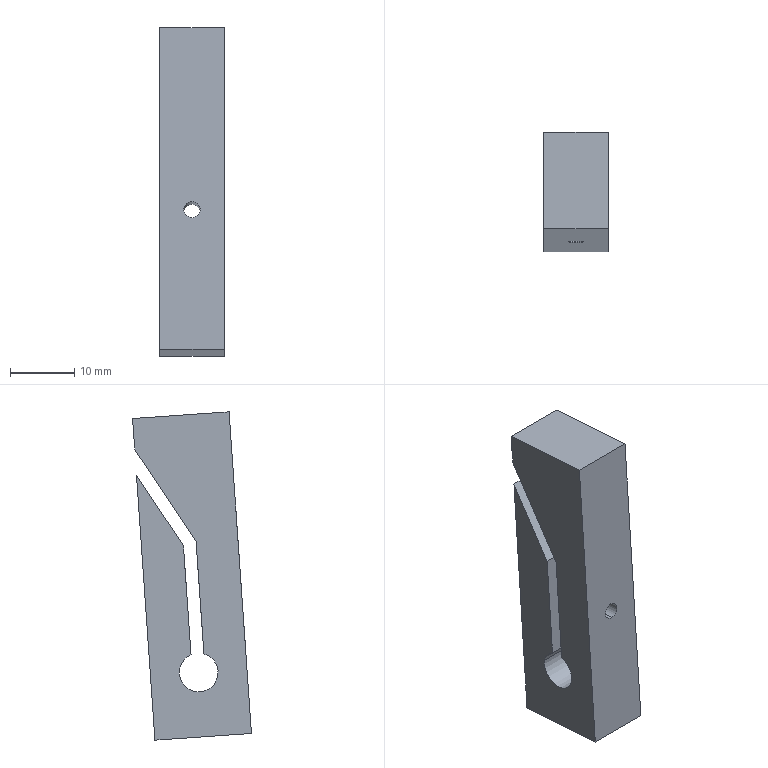Component | SolidWorks | Counterweight-1 | 1 solid | 23 faces | box 10 x 18.44 x 50.92 mm | volume 6250 mm3 | plane 13 | cylinder 8 | cone 2 | commonest cylinder face diameters 4 x3 6 x3 2.5 x2
build123d program:
from build123d import *

# Parameters (mm, degrees)
SKETCH2_R                    = 3
BOSS_EXTRUDE1_DEPTH          = 10
CUT_EXTRUDE_THIN1_DEPTH      = 48.843
CUT_EXTRUDE_THIN1_DEPTH_BACK = 10
CUT_EXTRUDE1_DEPTH           = 8
M3_TAPPED_HOLE1_D            = 2.5
M3_TAPPED_HOLE1_CSINK_D      = 3.05
M3_TAPPED_HOLE1_CSINK_ANGLE  = 90


with BuildPart() as part:
    # Sketch2 → Boss-Extrude1 (new body)
    with BuildSketch(Plane.XY):
        Polygon((1.842, 36.796), (-9.381, -11.928), (-23.998, -8.561), (-12.775, 40.163), align=None)
        with Locations((-14.445, -0.5)):
            Circle(SKETCH2_R, mode=Mode.SUBTRACT)
    extrude(amount=-BOSS_EXTRUDE1_DEPTH)

    # Sketch3 → Cut-Extrude-Thin1 (cut, two sides: drawn at the far end of the back side and taken through both)
    with BuildSketch(Plane.XY.offset(-CUT_EXTRUDE_THIN1_DEPTH_BACK)):
        Polygon((-13.47, -0.7245), (-9.04, 18.508), (2.431, 31.023), (0.9571, 32.375), (-10.871, 19.471), (-15.419, -0.2755), align=None)
    extrude(amount=CUT_EXTRUDE_THIN1_DEPTH + CUT_EXTRUDE_THIN1_DEPTH_BACK, mode=Mode.SUBTRACT)

    # Sketch4 → Cut-Extrude1 (cut)
    with BuildSketch(Plane(origin=(-6.299, 1.451, 0), x_dir=(0, 0, -1), z_dir=(0.9745, -0.2245, 0))):
        with BuildLine():
            Line((7, 12.007), (7, 4.007))
            ThreePointArc((7, 4.007), (5, 2.007), (3, 4.007))
            Line((3, 4.007), (3, 12.007))
            ThreePointArc((3, 12.007), (5, 14.007), (7, 12.007))
        make_face()
    extrude(amount=-CUT_EXTRUDE1_DEPTH, mode=Mode.SUBTRACT)

    # M3 Tapped Hole1 (through all)
    with Locations(Plane(origin=(-14.582, 3.359, 0), x_dir=(0, 0, -1), z_dir=(0.9745, -0.2245, 0))):
        with Locations((5, 8.007)):
            CounterSinkHole(M3_TAPPED_HOLE1_D / 2, M3_TAPPED_HOLE1_CSINK_D / 2, counter_sink_angle=M3_TAPPED_HOLE1_CSINK_ANGLE)


solid = part.part

# Placed as in the assembly
solid = solid.moved(Location((-513.446, 26.616, 404.902), (98.98, 90, 0)))
STEP:
#1=COLOUR_RGB('',0.7922,0.8196,0.9333);
#2=FILL_AREA_STYLE_COLOUR('',#1);
#3=FILL_AREA_STYLE('',(#2));
#4=SURFACE_STYLE_FILL_AREA(#3);
#5=SURFACE_SIDE_STYLE('',(#4));
#6=SURFACE_STYLE_USAGE(.BOTH.,#5);
#7=PRESENTATION_STYLE_ASSIGNMENT((#6));
#8=CARTESIAN_POINT('',(-20.411,0.4679,16.248));
#9=VERTEX_POINT('',#8);
#10=CARTESIAN_POINT('',(-20.411,0.4747,16.346));
#11=VERTEX_POINT('',#10);
#12=CARTESIAN_POINT('',(-20.411,0.4713,16.297));
#13=DIRECTION('',(-0.,0.9976,-0.0696));
#14=DIRECTION('',(0.,0.0696,0.9976));
#15=AXIS2_PLACEMENT_3D('',#12,#13,#14);
#16=CIRCLE('',#15,0.04921);
#17=EDGE_CURVE('',#9,#11,#16,.T.);
#18=ORIENTED_EDGE('',*,*,#17,.F.);
#19=CARTESIAN_POINT('',(-20.411,0.4779,16.237));
#20=VERTEX_POINT('',#19);
#21=CARTESIAN_POINT('',(-20.411,0.4779,16.237));
#22=DIRECTION('',(-0.,0.6562,-0.7546));
#23=VECTOR('',#22,39.37);
#24=LINE('',#21,#23);
#25=EDGE_CURVE('',#9,#20,#24,.T.);
#26=ORIENTED_EDGE('',*,*,#25,.T.);
#27=CARTESIAN_POINT('',(-20.411,0.4863,16.356));
#28=VERTEX_POINT('',#27);
#29=CARTESIAN_POINT('',(-20.411,0.4821,16.296));
#30=DIRECTION('',(-0.,0.9976,-0.0696));
#31=DIRECTION('',(0.,0.0696,0.9976));
#32=AXIS2_PLACEMENT_3D('',#29,#30,#31);
#33=CIRCLE('',#32,0.06004);
#34=EDGE_CURVE('',#20,#28,#33,.T.);
#35=ORIENTED_EDGE('',*,*,#34,.T.);
#36=CARTESIAN_POINT('',(-20.411,0.4863,16.356));
#37=DIRECTION('',(0.,0.7546,0.6562));
#38=VECTOR('',#37,39.37);
#39=LINE('',#36,#38);
#40=EDGE_CURVE('',#11,#28,#39,.T.);
#41=ORIENTED_EDGE('',*,*,#40,.F.);
#42=EDGE_LOOP('',(#18,#26,#35,#41));
#43=FACE_OUTER_BOUND('',#42,.T.);
#44=CARTESIAN_POINT('',(-20.411,0.4821,16.296));
#45=DIRECTION('',(-0.,0.9976,-0.0696));
#46=DIRECTION('',(0.,0.0696,0.9976));
#47=AXIS2_PLACEMENT_3D('',#44,#45,#46);
#48=CONICAL_SURFACE('',#47,0.06004,0.7854);
#49=ADVANCED_FACE('',(#43),#48,.F.);
#50=CARTESIAN_POINT('',(-20.411,0.2303,16.363));
#51=VERTEX_POINT('',#50);
#52=CARTESIAN_POINT('',(-20.411,0.2234,16.265));
#53=VERTEX_POINT('',#52);
#54=CARTESIAN_POINT('',(-20.411,0.2268,16.314));
#55=DIRECTION('',(0.,-0.9976,0.0696));
#56=DIRECTION('',(0.,-0.0696,-0.9976));
#57=AXIS2_PLACEMENT_3D('',#54,#55,#56);
#58=CIRCLE('',#57,0.04921);
#59=EDGE_CURVE('',#51,#53,#58,.T.);
#60=ORIENTED_EDGE('',*,*,#59,.T.);
#61=CARTESIAN_POINT('',(-20.411,0.4787,16.247));
#62=DIRECTION('',(-0.,0.9976,-0.0696));
#63=VECTOR('',#62,39.37);
#64=LINE('',#61,#63);
#65=EDGE_CURVE('',#53,#9,#64,.T.);
#66=ORIENTED_EDGE('',*,*,#65,.T.);
#67=ORIENTED_EDGE('',*,*,#17,.T.);
#68=CARTESIAN_POINT('',(-20.411,0.4855,16.346));
#69=DIRECTION('',(-0.,0.9976,-0.0696));
#70=VECTOR('',#69,39.37);
#71=LINE('',#68,#70);
#72=EDGE_CURVE('',#51,#11,#71,.T.);
#73=ORIENTED_EDGE('',*,*,#72,.F.);
#74=EDGE_LOOP('',(#60,#66,#67,#73));
#75=FACE_OUTER_BOUND('',#74,.T.);
#76=CARTESIAN_POINT('',(-20.411,0.4821,16.296));
#77=DIRECTION('',(-0.,0.9976,-0.0696));
#78=DIRECTION('',(0.,0.0696,0.9976));
#79=AXIS2_PLACEMENT_3D('',#76,#77,#78);
#80=CYLINDRICAL_SURFACE('',#79,0.04921);
#81=ADVANCED_FACE('',(#75),#80,.F.);
#82=CARTESIAN_POINT('',(-20.333,0.5716,16.448));
#83=VERTEX_POINT('',#82);
#84=CARTESIAN_POINT('',(-20.411,0.5771,16.527));
#85=VERTEX_POINT('',#84);
#86=CARTESIAN_POINT('',(-20.411,0.5716,16.448));
#87=DIRECTION('',(0.,-0.9976,0.0696));
#88=DIRECTION('',(0.,-0.0696,-0.9976));
#89=AXIS2_PLACEMENT_3D('',#86,#87,#88);
#90=CIRCLE('',#89,0.07874);
#91=EDGE_CURVE('',#83,#85,#90,.T.);
#92=ORIENTED_EDGE('',*,*,#91,.T.);
#93=CARTESIAN_POINT('',(-20.411,0.8324,16.509));
#94=VERTEX_POINT('',#93);
#95=CARTESIAN_POINT('',(-20.411,0.5182,16.531));
#96=DIRECTION('',(-0.,0.9976,-0.0696));
#97=VECTOR('',#96,39.37);
#98=LINE('',#95,#97);
#99=EDGE_CURVE('',#85,#94,#98,.T.);
#100=ORIENTED_EDGE('',*,*,#99,.T.);
#101=CARTESIAN_POINT('',(-20.333,0.8269,16.43));
#102=VERTEX_POINT('',#101);
#103=CARTESIAN_POINT('',(-20.411,0.8269,16.43));
#104=DIRECTION('',(-0.,0.9976,-0.0696));
#105=DIRECTION('',(0.,0.0696,0.9976));
#106=AXIS2_PLACEMENT_3D('',#103,#104,#105);
#107=CIRCLE('',#106,0.07874);
#108=EDGE_CURVE('',#94,#102,#107,.T.);
#109=ORIENTED_EDGE('',*,*,#108,.T.);
#110=CARTESIAN_POINT('',(-20.333,0.5127,16.452));
#111=DIRECTION('',(-0.,0.9976,-0.0696));
#112=VECTOR('',#111,39.37);
#113=LINE('',#110,#112);
#114=EDGE_CURVE('',#83,#102,#113,.T.);
#115=ORIENTED_EDGE('',*,*,#114,.F.);
#116=EDGE_LOOP('',(#92,#100,#109,#115));
#117=FACE_OUTER_BOUND('',#116,.T.);
#118=CARTESIAN_POINT('',(-20.411,0.5127,16.452));
#119=DIRECTION('',(-0.,0.9976,-0.0696));
#120=DIRECTION('',(0.,0.0696,0.9976));
#121=AXIS2_PLACEMENT_3D('',#118,#119,#120);
#122=CYLINDRICAL_SURFACE('',#121,0.07874);
#123=ADVANCED_FACE('',(#117),#122,.F.);
#124=CARTESIAN_POINT('',(-20.608,0.3726,15.814));
#125=VERTEX_POINT('',#124);
#126=CARTESIAN_POINT('',(-20.608,0.6059,15.851));
#127=VERTEX_POINT('',#126);
#128=CARTESIAN_POINT('',(-20.608,0.4892,15.833));
#129=DIRECTION('',(1.,-0.,-0.));
#130=DIRECTION('',(0.,0.9877,0.1561));
#131=AXIS2_PLACEMENT_3D('',#128,#129,#130);
#132=CIRCLE('',#131,0.1181);
#133=EDGE_CURVE('',#125,#127,#132,.T.);
#134=ORIENTED_EDGE('',*,*,#133,.F.);
#135=CARTESIAN_POINT('',(-20.214,0.3726,15.814));
#136=VERTEX_POINT('',#135);
#137=CARTESIAN_POINT('',(-20.608,0.3726,15.814));
#138=DIRECTION('',(1.,-0.,-0.));
#139=VECTOR('',#138,39.37);
#140=LINE('',#137,#139);
#141=EDGE_CURVE('',#125,#136,#140,.T.);
#142=ORIENTED_EDGE('',*,*,#141,.T.);
#143=CARTESIAN_POINT('',(-20.214,0.6059,15.851));
#144=VERTEX_POINT('',#143);
#145=CARTESIAN_POINT('',(-20.214,0.4892,15.833));
#146=DIRECTION('',(1.,-0.,-0.));
#147=DIRECTION('',(0.,0.9877,0.1561));
#148=AXIS2_PLACEMENT_3D('',#145,#146,#147);
#149=CIRCLE('',#148,0.1181);
#150=EDGE_CURVE('',#136,#144,#149,.T.);
#151=ORIENTED_EDGE('',*,*,#150,.T.);
#152=CARTESIAN_POINT('',(-20.608,0.6059,15.851));
#153=DIRECTION('',(1.,-0.,-0.));
#154=VECTOR('',#153,39.37);
#155=LINE('',#152,#154);
#156=EDGE_CURVE('',#127,#144,#155,.T.);
#157=ORIENTED_EDGE('',*,*,#156,.F.);
#158=EDGE_LOOP('',(#134,#142,#151,#157));
#159=FACE_OUTER_BOUND('',#158,.T.);
#160=CARTESIAN_POINT('',(-20.608,0.4892,15.833));
#161=DIRECTION('',(1.,-0.,-0.));
#162=DIRECTION('',(0.,0.9877,0.1561));
#163=AXIS2_PLACEMENT_3D('',#160,#161,#162);
#164=CYLINDRICAL_SURFACE('',#163,0.1181);
#165=ADVANCED_FACE('',(#159),#164,.F.);
#166=CARTESIAN_POINT('',(-20.608,0.5363,15.941));
#167=VERTEX_POINT('',#166);
#168=CARTESIAN_POINT('',(-20.608,0.4892,15.833));
#169=DIRECTION('',(1.,-0.,-0.));
#170=DIRECTION('',(0.,0.9877,0.1561));
#171=AXIS2_PLACEMENT_3D('',#168,#169,#170);
#172=CIRCLE('',#171,0.1181);
#173=EDGE_CURVE('',#127,#167,#172,.T.);
#174=ORIENTED_EDGE('',*,*,#173,.F.);
#175=ORIENTED_EDGE('',*,*,#156,.T.);
#176=CARTESIAN_POINT('',(-20.214,0.5363,15.941));
#177=VERTEX_POINT('',#176);
#178=CARTESIAN_POINT('',(-20.214,0.4892,15.833));
#179=DIRECTION('',(1.,-0.,-0.));
#180=DIRECTION('',(0.,0.9877,0.1561));
#181=AXIS2_PLACEMENT_3D('',#178,#179,#180);
#182=CIRCLE('',#181,0.1181);
#183=EDGE_CURVE('',#144,#177,#182,.T.);
#184=ORIENTED_EDGE('',*,*,#183,.T.);
#185=CARTESIAN_POINT('',(-20.608,0.5363,15.941));
#186=DIRECTION('',(1.,-0.,-0.));
#187=VECTOR('',#186,39.37);
#188=LINE('',#185,#187);
#189=EDGE_CURVE('',#167,#177,#188,.T.);
#190=ORIENTED_EDGE('',*,*,#189,.F.);
#191=EDGE_LOOP('',(#174,#175,#184,#190));
#192=FACE_OUTER_BOUND('',#191,.T.);
#193=CARTESIAN_POINT('',(-20.608,0.4892,15.833));
#194=DIRECTION('',(1.,-0.,-0.));
#195=DIRECTION('',(0.,0.9877,0.1561));
#196=AXIS2_PLACEMENT_3D('',#193,#194,#195);
#197=CYLINDRICAL_SURFACE('',#196,0.1181);
#198=ADVANCED_FACE('',(#192),#197,.F.);
#199=CARTESIAN_POINT('',(-20.49,0.8269,16.43));
#200=VERTEX_POINT('',#199);
#201=CARTESIAN_POINT('',(-20.411,0.8269,16.43));
#202=DIRECTION('',(-0.,0.9976,-0.0696));
#203=DIRECTION('',(0.,0.0696,0.9976));
#204=AXIS2_PLACEMENT_3D('',#201,#202,#203);
#205=CIRCLE('',#204,0.07874);
#206=EDGE_CURVE('',#200,#94,#205,.T.);
#207=ORIENTED_EDGE('',*,*,#206,.F.);
#208=CARTESIAN_POINT('',(-20.49,0.805,16.116));
#209=VERTEX_POINT('',#208);
#210=CARTESIAN_POINT('',(-20.49,0.8269,16.43));
#211=DIRECTION('',(0.,0.0696,0.9976));
#212=VECTOR('',#211,39.37);
#213=LINE('',#210,#212);
#214=EDGE_CURVE('',#209,#200,#213,.T.);
#215=ORIENTED_EDGE('',*,*,#214,.F.);
#216=CARTESIAN_POINT('',(-20.333,0.805,16.116));
#217=VERTEX_POINT('',#216);
#218=CARTESIAN_POINT('',(-20.411,0.805,16.116));
#219=DIRECTION('',(-0.,0.9976,-0.0696));
#220=DIRECTION('',(0.,0.0696,0.9976));
#221=AXIS2_PLACEMENT_3D('',#218,#219,#220);
#222=CIRCLE('',#221,0.07874);
#223=EDGE_CURVE('',#217,#209,#222,.T.);
#224=ORIENTED_EDGE('',*,*,#223,.F.);
#225=CARTESIAN_POINT('',(-20.333,0.8269,16.43));
#226=DIRECTION('',(-0.,-0.0696,-0.9976));
#227=VECTOR('',#226,39.37);
#228=LINE('',#225,#227);
#229=EDGE_CURVE('',#102,#217,#228,.T.);
#230=ORIENTED_EDGE('',*,*,#229,.F.);
#231=ORIENTED_EDGE('',*,*,#108,.F.);
#232=EDGE_LOOP('',(#207,#215,#224,#230,#231));
#233=FACE_BOUND('',#232,.T.);
#234=CARTESIAN_POINT('',(-20.608,0.7564,15.42));
#235=VERTEX_POINT('',#234);
#236=CARTESIAN_POINT('',(-20.608,0.8693,17.038));
#237=VERTEX_POINT('',#236);
#238=CARTESIAN_POINT('',(-20.608,0.8934,17.383));
#239=DIRECTION('',(0.,0.0696,0.9976));
#240=VECTOR('',#239,39.37);
#241=LINE('',#238,#240);
#242=EDGE_CURVE('',#235,#237,#241,.T.);
#243=ORIENTED_EDGE('',*,*,#242,.T.);
#244=CARTESIAN_POINT('',(-20.214,0.8693,17.038));
#245=VERTEX_POINT('',#244);
#246=CARTESIAN_POINT('',(-20.608,0.8693,17.038));
#247=DIRECTION('',(1.,-0.,-0.));
#248=VECTOR('',#247,39.37);
#249=LINE('',#246,#248);
#250=EDGE_CURVE('',#237,#245,#249,.T.);
#251=ORIENTED_EDGE('',*,*,#250,.T.);
#252=CARTESIAN_POINT('',(-20.214,0.7564,15.42));
#253=VERTEX_POINT('',#252);
#254=CARTESIAN_POINT('',(-20.214,0.8934,17.383));
#255=DIRECTION('',(0.,0.0696,0.9976));
#256=VECTOR('',#255,39.37);
#257=LINE('',#254,#256);
#258=EDGE_CURVE('',#253,#245,#257,.T.);
#259=ORIENTED_EDGE('',*,*,#258,.F.);
#260=CARTESIAN_POINT('',(-20.608,0.7564,15.42));
#261=DIRECTION('',(1.,-0.,-0.));
#262=VECTOR('',#261,39.37);
#263=LINE('',#260,#262);
#264=EDGE_CURVE('',#235,#253,#263,.T.);
#265=ORIENTED_EDGE('',*,*,#264,.F.);
#266=EDGE_LOOP('',(#243,#251,#259,#265));
#267=FACE_OUTER_BOUND('',#266,.T.);
#268=CARTESIAN_POINT('',(-20.608,0.8934,17.383));
#269=DIRECTION('',(-0.,0.9976,-0.0696));
#270=DIRECTION('',(0.,0.0696,0.9976));
#271=AXIS2_PLACEMENT_3D('',#268,#269,#270);
#272=PLANE('',#271);
#273=ADVANCED_FACE('',(#233,#267),#272,.T.);
#274=CARTESIAN_POINT('',(-20.214,0.8934,17.383));
#275=VERTEX_POINT('',#274);
#276=CARTESIAN_POINT('',(-20.214,0.3043,17.424));
#277=VERTEX_POINT('',#276);
#278=CARTESIAN_POINT('',(-20.214,0.3043,17.424));
#279=DIRECTION('',(0.,-0.9976,0.0696));
#280=VECTOR('',#279,39.37);
#281=LINE('',#278,#280);
#282=EDGE_CURVE('',#275,#277,#281,.T.);
#283=ORIENTED_EDGE('',*,*,#282,.F.);
#284=CARTESIAN_POINT('',(-20.608,0.8934,17.383));
#285=VERTEX_POINT('',#284);
#286=CARTESIAN_POINT('',(-20.608,0.8934,17.383));
#287=DIRECTION('',(1.,-0.,-0.));
#288=VECTOR('',#287,39.37);
#289=LINE('',#286,#288);
#290=EDGE_CURVE('',#285,#275,#289,.T.);
#291=ORIENTED_EDGE('',*,*,#290,.F.);
#292=CARTESIAN_POINT('',(-20.608,0.3043,17.424));
#293=VERTEX_POINT('',#292);
#294=CARTESIAN_POINT('',(-20.608,0.3043,17.424));
#295=DIRECTION('',(0.,-0.9976,0.0696));
#296=VECTOR('',#295,39.37);
#297=LINE('',#294,#296);
#298=EDGE_CURVE('',#285,#293,#297,.T.);
#299=ORIENTED_EDGE('',*,*,#298,.T.);
#300=CARTESIAN_POINT('',(-20.608,0.3043,17.424));
#301=DIRECTION('',(1.,-0.,-0.));
#302=VECTOR('',#301,39.37);
#303=LINE('',#300,#302);
#304=EDGE_CURVE('',#293,#277,#303,.T.);
#305=ORIENTED_EDGE('',*,*,#304,.T.);
#306=EDGE_LOOP('',(#283,#291,#299,#305));
#307=FACE_OUTER_BOUND('',#306,.T.);
#308=CARTESIAN_POINT('',(-20.608,0.3043,17.424));
#309=DIRECTION('',(0.,0.0696,0.9976));
#310=DIRECTION('',(0.,-0.9976,0.0696));
#311=AXIS2_PLACEMENT_3D('',#308,#309,#310);
#312=PLANE('',#311);
#313=ADVANCED_FACE('',(#307),#312,.T.);
#314=CARTESIAN_POINT('',(-20.608,0.8804,17.197));
#315=VERTEX_POINT('',#314);
#316=CARTESIAN_POINT('',(-20.214,0.8804,17.197));
#317=VERTEX_POINT('',#316);
#318=CARTESIAN_POINT('',(-20.608,0.8804,17.197));
#319=DIRECTION('',(1.,-0.,-0.));
#320=VECTOR('',#319,39.37);
#321=LINE('',#318,#320);
#322=EDGE_CURVE('',#315,#317,#321,.T.);
#323=ORIENTED_EDGE('',*,*,#322,.F.);
#324=CARTESIAN_POINT('',(-20.608,0.8934,17.383));
#325=DIRECTION('',(0.,0.0696,0.9976));
#326=VECTOR('',#325,39.37);
#327=LINE('',#324,#326);
#328=EDGE_CURVE('',#315,#285,#327,.T.);
#329=ORIENTED_EDGE('',*,*,#328,.T.);
#330=ORIENTED_EDGE('',*,*,#290,.T.);
#331=CARTESIAN_POINT('',(-20.214,0.8934,17.383));
#332=DIRECTION('',(0.,0.0696,0.9976));
#333=VECTOR('',#332,39.37);
#334=LINE('',#331,#333);
#335=EDGE_CURVE('',#317,#275,#334,.T.);
#336=ORIENTED_EDGE('',*,*,#335,.F.);
#337=EDGE_LOOP('',(#323,#329,#330,#336));
#338=FACE_OUTER_BOUND('',#337,.T.);
#339=CARTESIAN_POINT('',(-20.608,0.8934,17.383));
#340=DIRECTION('',(-0.,0.9976,-0.0696));
#341=DIRECTION('',(0.,0.0696,0.9976));
#342=AXIS2_PLACEMENT_3D('',#339,#340,#341);
#343=PLANE('',#342);
#344=ADVANCED_FACE('',(#338),#343,.T.);
#345=CARTESIAN_POINT('',(-20.214,0.1673,15.461));
#346=VERTEX_POINT('',#345);
#347=CARTESIAN_POINT('',(-20.214,0.7564,15.42));
#348=DIRECTION('',(-0.,0.9976,-0.0696));
#349=VECTOR('',#348,39.37);
#350=LINE('',#347,#349);
#351=EDGE_CURVE('',#346,#253,#350,.T.);
#352=ORIENTED_EDGE('',*,*,#351,.F.);
#353=CARTESIAN_POINT('',(-20.608,0.1673,15.461));
#354=VERTEX_POINT('',#353);
#355=CARTESIAN_POINT('',(-20.608,0.1673,15.461));
#356=DIRECTION('',(1.,-0.,-0.));
#357=VECTOR('',#356,39.37);
#358=LINE('',#355,#357);
#359=EDGE_CURVE('',#354,#346,#358,.T.);
#360=ORIENTED_EDGE('',*,*,#359,.F.);
#361=CARTESIAN_POINT('',(-20.608,0.7564,15.42));
#362=DIRECTION('',(-0.,0.9976,-0.0696));
#363=VECTOR('',#362,39.37);
#364=LINE('',#361,#363);
#365=EDGE_CURVE('',#354,#235,#364,.T.);
#366=ORIENTED_EDGE('',*,*,#365,.T.);
#367=ORIENTED_EDGE('',*,*,#264,.T.);
#368=EDGE_LOOP('',(#352,#360,#366,#367));
#369=FACE_OUTER_BOUND('',#368,.T.);
#370=CARTESIAN_POINT('',(-20.608,0.7564,15.42));
#371=DIRECTION('',(-0.,-0.0696,-0.9976));
#372=DIRECTION('',(-0.,0.9976,-0.0696));
#373=AXIS2_PLACEMENT_3D('',#370,#371,#372);
#374=PLANE('',#373);
#375=ADVANCED_FACE('',(#369),#374,.T.);
#376=ORIENTED_EDGE('',*,*,#59,.F.);
#377=CARTESIAN_POINT('',(-20.411,0.2268,16.314));
#378=DIRECTION('',(0.,-0.9976,0.0696));
#379=DIRECTION('',(0.,-0.0696,-0.9976));
#380=AXIS2_PLACEMENT_3D('',#377,#378,#379);
#381=CIRCLE('',#380,0.04921);
#382=EDGE_CURVE('',#53,#51,#381,.T.);
#383=ORIENTED_EDGE('',*,*,#382,.F.);
#384=EDGE_LOOP('',(#376,#383));
#385=FACE_BOUND('',#384,.T.);
#386=CARTESIAN_POINT('',(-20.214,0.1673,15.461));
#387=DIRECTION('',(-0.,-0.0696,-0.9976));
#388=VECTOR('',#387,39.37);
#389=LINE('',#386,#388);
#390=EDGE_CURVE('',#277,#346,#389,.T.);
#391=ORIENTED_EDGE('',*,*,#390,.F.);
#392=ORIENTED_EDGE('',*,*,#304,.F.);
#393=CARTESIAN_POINT('',(-20.608,0.1673,15.461));
#394=DIRECTION('',(-0.,-0.0696,-0.9976));
#395=VECTOR('',#394,39.37);
#396=LINE('',#393,#395);
#397=EDGE_CURVE('',#293,#354,#396,.T.);
#398=ORIENTED_EDGE('',*,*,#397,.T.);
#399=ORIENTED_EDGE('',*,*,#359,.T.);
#400=EDGE_LOOP('',(#391,#392,#398,#399));
#401=FACE_OUTER_BOUND('',#400,.T.);
#402=CARTESIAN_POINT('',(-20.608,0.1673,15.461));
#403=DIRECTION('',(0.,-0.9976,0.0696));
#404=DIRECTION('',(-0.,-0.0696,-0.9976));
#405=AXIS2_PLACEMENT_3D('',#402,#403,#404);
#406=PLANE('',#405);
#407=ADVANCED_FACE('',(#385,#401),#406,.T.);
#408=CARTESIAN_POINT('',(-20.608,0.5055,16.631));
#409=VERTEX_POINT('',#408);
#410=CARTESIAN_POINT('',(-20.608,0.5112,16.64));
#411=DIRECTION('',(0.,0.5524,0.8336));
#412=VECTOR('',#411,39.37);
#413=LINE('',#410,#412);
#414=EDGE_CURVE('',#409,#315,#413,.T.);
#415=ORIENTED_EDGE('',*,*,#414,.F.);
#416=CARTESIAN_POINT('',(-20.608,0.4577,15.947));
#417=VERTEX_POINT('',#416);
#418=CARTESIAN_POINT('',(-20.608,0.45,15.836));
#419=DIRECTION('',(0.,0.0696,0.9976));
#420=VECTOR('',#419,39.37);
#421=LINE('',#418,#420);
#422=EDGE_CURVE('',#417,#409,#421,.T.);
#423=ORIENTED_EDGE('',*,*,#422,.F.);
#424=CARTESIAN_POINT('',(-20.608,0.4892,15.833));
#425=DIRECTION('',(1.,-0.,-0.));
#426=DIRECTION('',(0.,0.9877,0.1561));
#427=AXIS2_PLACEMENT_3D('',#424,#425,#426);
#428=CIRCLE('',#427,0.1181);
#429=EDGE_CURVE('',#417,#125,#428,.T.);
#430=ORIENTED_EDGE('',*,*,#429,.T.);
#431=ORIENTED_EDGE('',*,*,#133,.T.);
#432=ORIENTED_EDGE('',*,*,#173,.T.);
#433=CARTESIAN_POINT('',(-20.608,0.5826,16.605));
#434=VERTEX_POINT('',#433);
#435=CARTESIAN_POINT('',(-20.608,0.5285,15.83));
#436=DIRECTION('',(0.,0.0696,0.9976));
#437=VECTOR('',#436,39.37);
#438=LINE('',#435,#437);
#439=EDGE_CURVE('',#167,#434,#438,.T.);
#440=ORIENTED_EDGE('',*,*,#439,.T.);
#441=CARTESIAN_POINT('',(-20.608,0.5769,16.597));
#442=DIRECTION('',(0.,0.5524,0.8336));
#443=VECTOR('',#442,39.37);
#444=LINE('',#441,#443);
#445=EDGE_CURVE('',#434,#237,#444,.T.);
#446=ORIENTED_EDGE('',*,*,#445,.T.);
#447=ORIENTED_EDGE('',*,*,#242,.F.);
#448=ORIENTED_EDGE('',*,*,#365,.F.);
#449=ORIENTED_EDGE('',*,*,#397,.F.);
#450=ORIENTED_EDGE('',*,*,#298,.F.);
#451=ORIENTED_EDGE('',*,*,#328,.F.);
#452=EDGE_LOOP('',(#415,#423,#430,#431,#432,#440,#446,#447,#448,#449,#450,#451));
#453=FACE_OUTER_BOUND('',#452,.T.);
#454=CARTESIAN_POINT('',(-20.608,1.048,15.941));
#455=DIRECTION('',(-1.,0.,0.));
#456=DIRECTION('',(-0.,-0.9877,-0.1561));
#457=AXIS2_PLACEMENT_3D('',#454,#455,#456);
#458=PLANE('',#457);
#459=ADVANCED_FACE('',(#453),#458,.T.);
#460=CARTESIAN_POINT('',(-20.214,0.4577,15.947));
#461=VERTEX_POINT('',#460);
#462=CARTESIAN_POINT('',(-20.214,0.5055,16.631));
#463=VERTEX_POINT('',#462);
#464=CARTESIAN_POINT('',(-20.214,0.4602,15.982));
#465=DIRECTION('',(0.,0.0696,0.9976));
#466=VECTOR('',#465,39.37);
#467=LINE('',#464,#466);
#468=EDGE_CURVE('',#461,#463,#467,.T.);
#469=ORIENTED_EDGE('',*,*,#468,.T.);
#470=CARTESIAN_POINT('',(-20.214,0.3531,16.401));
#471=DIRECTION('',(0.,0.5524,0.8336));
#472=VECTOR('',#471,39.37);
#473=LINE('',#470,#472);
#474=EDGE_CURVE('',#463,#317,#473,.T.);
#475=ORIENTED_EDGE('',*,*,#474,.T.);
#476=ORIENTED_EDGE('',*,*,#335,.T.);
#477=ORIENTED_EDGE('',*,*,#282,.T.);
#478=ORIENTED_EDGE('',*,*,#390,.T.);
#479=ORIENTED_EDGE('',*,*,#351,.T.);
#480=ORIENTED_EDGE('',*,*,#258,.T.);
#481=CARTESIAN_POINT('',(-20.214,0.5826,16.605));
#482=VERTEX_POINT('',#481);
#483=CARTESIAN_POINT('',(-20.214,0.4187,16.358));
#484=DIRECTION('',(0.,0.5524,0.8336));
#485=VECTOR('',#484,39.37);
#486=LINE('',#483,#485);
#487=EDGE_CURVE('',#482,#245,#486,.T.);
#488=ORIENTED_EDGE('',*,*,#487,.F.);
#489=CARTESIAN_POINT('',(-20.214,0.5387,15.977));
#490=DIRECTION('',(0.,0.0696,0.9976));
#491=VECTOR('',#490,39.37);
#492=LINE('',#489,#491);
#493=EDGE_CURVE('',#177,#482,#492,.T.);
#494=ORIENTED_EDGE('',*,*,#493,.F.);
#495=ORIENTED_EDGE('',*,*,#183,.F.);
#496=ORIENTED_EDGE('',*,*,#150,.F.);
#497=CARTESIAN_POINT('',(-20.214,0.4892,15.833));
#498=DIRECTION('',(1.,-0.,-0.));
#499=DIRECTION('',(0.,0.9877,0.1561));
#500=AXIS2_PLACEMENT_3D('',#497,#498,#499);
#501=CIRCLE('',#500,0.1181);
#502=EDGE_CURVE('',#461,#136,#501,.T.);
#503=ORIENTED_EDGE('',*,*,#502,.F.);
#504=EDGE_LOOP('',(#469,#475,#476,#477,#478,#479,#480,#488,#494,#495,#496,#503));
#505=FACE_OUTER_BOUND('',#504,.T.);
#506=CARTESIAN_POINT('',(-20.214,1.048,15.941));
#507=DIRECTION('',(-1.,0.,0.));
#508=DIRECTION('',(-0.,-0.9877,-0.1561));
#509=AXIS2_PLACEMENT_3D('',#506,#507,#508);
#510=PLANE('',#509);
#511=ADVANCED_FACE('',(#505),#510,.F.);
#512=ORIENTED_EDGE('',*,*,#141,.F.);
#513=ORIENTED_EDGE('',*,*,#429,.F.);
#514=CARTESIAN_POINT('',(-20.608,0.4577,15.947));
#515=DIRECTION('',(1.,-0.,-0.));
#516=VECTOR('',#515,39.37);
#517=LINE('',#514,#516);
#518=EDGE_CURVE('',#417,#461,#517,.T.);
#519=ORIENTED_EDGE('',*,*,#518,.T.);
#520=ORIENTED_EDGE('',*,*,#502,.T.);
#521=EDGE_LOOP('',(#512,#513,#519,#520));
#522=FACE_OUTER_BOUND('',#521,.T.);
#523=CARTESIAN_POINT('',(-20.608,0.4892,15.833));
#524=DIRECTION('',(1.,-0.,-0.));
#525=DIRECTION('',(0.,0.9877,0.1561));
#526=AXIS2_PLACEMENT_3D('',#523,#524,#525);
#527=CYLINDRICAL_SURFACE('',#526,0.1181);
#528=ADVANCED_FACE('',(#522),#527,.F.);
#529=ORIENTED_EDGE('',*,*,#91,.F.);
#530=CARTESIAN_POINT('',(-20.333,0.5497,16.134));
#531=VERTEX_POINT('',#530);
#532=CARTESIAN_POINT('',(-20.333,0.5285,15.83));
#533=DIRECTION('',(0.,0.0696,0.9976));
#534=VECTOR('',#533,39.37);
#535=LINE('',#532,#534);
#536=EDGE_CURVE('',#531,#83,#535,.T.);
#537=ORIENTED_EDGE('',*,*,#536,.F.);
#538=CARTESIAN_POINT('',(-20.49,0.5497,16.134));
#539=VERTEX_POINT('',#538);
#540=CARTESIAN_POINT('',(-20.411,0.5497,16.134));
#541=DIRECTION('',(0.,-0.9976,0.0696));
#542=DIRECTION('',(0.,-0.0696,-0.9976));
#543=AXIS2_PLACEMENT_3D('',#540,#541,#542);
#544=CIRCLE('',#543,0.07874);
#545=EDGE_CURVE('',#539,#531,#544,.T.);
#546=ORIENTED_EDGE('',*,*,#545,.F.);
#547=CARTESIAN_POINT('',(-20.49,0.5716,16.448));
#548=VERTEX_POINT('',#547);
#549=CARTESIAN_POINT('',(-20.49,0.5285,15.83));
#550=DIRECTION('',(-0.,-0.0696,-0.9976));
#551=VECTOR('',#550,39.37);
#552=LINE('',#549,#551);
#553=EDGE_CURVE('',#548,#539,#552,.T.);
#554=ORIENTED_EDGE('',*,*,#553,.F.);
#555=CARTESIAN_POINT('',(-20.411,0.5716,16.448));
#556=DIRECTION('',(0.,-0.9976,0.0696));
#557=DIRECTION('',(0.,-0.0696,-0.9976));
#558=AXIS2_PLACEMENT_3D('',#555,#556,#557);
#559=CIRCLE('',#558,0.07874);
#560=EDGE_CURVE('',#85,#548,#559,.T.);
#561=ORIENTED_EDGE('',*,*,#560,.F.);
#562=EDGE_LOOP('',(#529,#537,#546,#554,#561));
#563=FACE_BOUND('',#562,.T.);
#564=ORIENTED_EDGE('',*,*,#493,.T.);
#565=CARTESIAN_POINT('',(-20.214,0.5826,16.605));
#566=DIRECTION('',(-1.,0.,0.));
#567=VECTOR('',#566,39.37);
#568=LINE('',#565,#567);
#569=EDGE_CURVE('',#482,#434,#568,.T.);
#570=ORIENTED_EDGE('',*,*,#569,.T.);
#571=ORIENTED_EDGE('',*,*,#439,.F.);
#572=ORIENTED_EDGE('',*,*,#189,.T.);
#573=EDGE_LOOP('',(#564,#570,#571,#572));
#574=FACE_OUTER_BOUND('',#573,.T.);
#575=CARTESIAN_POINT('',(-20.214,0.5285,15.83));
#576=DIRECTION('',(0.,-0.9976,0.0696));
#577=DIRECTION('',(-0.,-0.0696,-0.9976));
#578=AXIS2_PLACEMENT_3D('',#575,#576,#577);
#579=PLANE('',#578);
#580=ADVANCED_FACE('',(#563,#574),#579,.T.);
#581=ORIENTED_EDGE('',*,*,#445,.F.);
#582=ORIENTED_EDGE('',*,*,#569,.F.);
#583=ORIENTED_EDGE('',*,*,#487,.T.);
#584=ORIENTED_EDGE('',*,*,#250,.F.);
#585=EDGE_LOOP('',(#581,#582,#583,#584));
#586=FACE_OUTER_BOUND('',#585,.T.);
#587=CARTESIAN_POINT('',(-20.214,0.5769,16.597));
#588=DIRECTION('',(0.,-0.8336,0.5524));
#589=DIRECTION('',(-0.,-0.5524,-0.8336));
#590=AXIS2_PLACEMENT_3D('',#587,#588,#589);
#591=PLANE('',#590);
#592=ADVANCED_FACE('',(#586),#591,.T.);
#593=CARTESIAN_POINT('',(-20.411,0.4821,16.296));
#594=DIRECTION('',(-0.,0.9976,-0.0696));
#595=DIRECTION('',(0.,0.0696,0.9976));
#596=AXIS2_PLACEMENT_3D('',#593,#594,#595);
#597=CIRCLE('',#596,0.06004);
#598=EDGE_CURVE('',#28,#20,#597,.T.);
#599=ORIENTED_EDGE('',*,*,#598,.F.);
#600=ORIENTED_EDGE('',*,*,#34,.F.);
#601=EDGE_LOOP('',(#599,#600));
#602=FACE_BOUND('',#601,.T.);
#603=ORIENTED_EDGE('',*,*,#518,.F.);
#604=ORIENTED_EDGE('',*,*,#422,.T.);
#605=CARTESIAN_POINT('',(-20.214,0.5055,16.631));
#606=DIRECTION('',(-1.,0.,0.));
#607=VECTOR('',#606,39.37);
#608=LINE('',#605,#607);
#609=EDGE_CURVE('',#463,#409,#608,.T.);
#610=ORIENTED_EDGE('',*,*,#609,.F.);
#611=ORIENTED_EDGE('',*,*,#468,.F.);
#612=EDGE_LOOP('',(#603,#604,#610,#611));
#613=FACE_OUTER_BOUND('',#612,.T.);
#614=CARTESIAN_POINT('',(-20.214,0.45,15.836));
#615=DIRECTION('',(0.,-0.9976,0.0696));
#616=DIRECTION('',(-0.,-0.0696,-0.9976));
#617=AXIS2_PLACEMENT_3D('',#614,#615,#616);
#618=PLANE('',#617);
#619=ADVANCED_FACE('',(#602,#613),#618,.F.);
#620=ORIENTED_EDGE('',*,*,#322,.T.);
#621=ORIENTED_EDGE('',*,*,#474,.F.);
#622=ORIENTED_EDGE('',*,*,#609,.T.);
#623=ORIENTED_EDGE('',*,*,#414,.T.);
#624=EDGE_LOOP('',(#620,#621,#622,#623));
#625=FACE_OUTER_BOUND('',#624,.T.);
#626=CARTESIAN_POINT('',(-20.214,0.5112,16.64));
#627=DIRECTION('',(0.,-0.8336,0.5524));
#628=DIRECTION('',(-0.,-0.5524,-0.8336));
#629=AXIS2_PLACEMENT_3D('',#626,#627,#628);
#630=PLANE('',#629);
#631=ADVANCED_FACE('',(#625),#630,.F.);
#632=ORIENTED_EDGE('',*,*,#99,.F.);
#633=ORIENTED_EDGE('',*,*,#560,.T.);
#634=CARTESIAN_POINT('',(-20.49,0.5127,16.452));
#635=DIRECTION('',(-0.,0.9976,-0.0696));
#636=VECTOR('',#635,39.37);
#637=LINE('',#634,#636);
#638=EDGE_CURVE('',#548,#200,#637,.T.);
#639=ORIENTED_EDGE('',*,*,#638,.T.);
#640=ORIENTED_EDGE('',*,*,#206,.T.);
#641=EDGE_LOOP('',(#632,#633,#639,#640));
#642=FACE_OUTER_BOUND('',#641,.T.);
#643=CARTESIAN_POINT('',(-20.411,0.5127,16.452));
#644=DIRECTION('',(-0.,0.9976,-0.0696));
#645=DIRECTION('',(0.,0.0696,0.9976));
#646=AXIS2_PLACEMENT_3D('',#643,#644,#645);
#647=CYLINDRICAL_SURFACE('',#646,0.07874);
#648=ADVANCED_FACE('',(#642),#647,.F.);
#649=ORIENTED_EDGE('',*,*,#553,.T.);
#650=CARTESIAN_POINT('',(-20.49,0.4908,16.138));
#651=DIRECTION('',(-0.,0.9976,-0.0696));
#652=VECTOR('',#651,39.37);
#653=LINE('',#650,#652);
#654=EDGE_CURVE('',#539,#209,#653,.T.);
#655=ORIENTED_EDGE('',*,*,#654,.T.);
#656=ORIENTED_EDGE('',*,*,#214,.T.);
#657=ORIENTED_EDGE('',*,*,#638,.F.);
#658=EDGE_LOOP('',(#649,#655,#656,#657));
#659=FACE_OUTER_BOUND('',#658,.T.);
#660=CARTESIAN_POINT('',(-20.49,0.5127,16.452));
#661=DIRECTION('',(-1.,0.,0.));
#662=DIRECTION('',(-0.,-0.9877,-0.1561));
#663=AXIS2_PLACEMENT_3D('',#660,#661,#662);
#664=PLANE('',#663);
#665=ADVANCED_FACE('',(#659),#664,.F.);
#666=ORIENTED_EDGE('',*,*,#545,.T.);
#667=CARTESIAN_POINT('',(-20.333,0.4908,16.138));
#668=DIRECTION('',(-0.,0.9976,-0.0696));
#669=VECTOR('',#668,39.37);
#670=LINE('',#667,#669);
#671=EDGE_CURVE('',#531,#217,#670,.T.);
#672=ORIENTED_EDGE('',*,*,#671,.T.);
#673=ORIENTED_EDGE('',*,*,#223,.T.);
#674=ORIENTED_EDGE('',*,*,#654,.F.);
#675=EDGE_LOOP('',(#666,#672,#673,#674));
#676=FACE_OUTER_BOUND('',#675,.T.);
#677=CARTESIAN_POINT('',(-20.411,0.4908,16.138));
#678=DIRECTION('',(-0.,0.9976,-0.0696));
#679=DIRECTION('',(0.,0.0696,0.9976));
#680=AXIS2_PLACEMENT_3D('',#677,#678,#679);
#681=CYLINDRICAL_SURFACE('',#680,0.07874);
#682=ADVANCED_FACE('',(#676),#681,.F.);
#683=ORIENTED_EDGE('',*,*,#536,.T.);
#684=ORIENTED_EDGE('',*,*,#114,.T.);
#685=ORIENTED_EDGE('',*,*,#229,.T.);
#686=ORIENTED_EDGE('',*,*,#671,.F.);
#687=EDGE_LOOP('',(#683,#684,#685,#686));
#688=FACE_OUTER_BOUND('',#687,.T.);
#689=CARTESIAN_POINT('',(-20.333,0.5127,16.452));
#690=DIRECTION('',(1.,-0.,-0.));
#691=DIRECTION('',(-0.,0.1561,-0.9877));
#692=AXIS2_PLACEMENT_3D('',#689,#690,#691);
#693=PLANE('',#692);
#694=ADVANCED_FACE('',(#688),#693,.F.);
#695=ORIENTED_EDGE('',*,*,#65,.F.);
#696=ORIENTED_EDGE('',*,*,#382,.T.);
#697=ORIENTED_EDGE('',*,*,#72,.T.);
#698=CARTESIAN_POINT('',(-20.411,0.4713,16.297));
#699=DIRECTION('',(-0.,0.9976,-0.0696));
#700=DIRECTION('',(0.,0.0696,0.9976));
#701=AXIS2_PLACEMENT_3D('',#698,#699,#700);
#702=CIRCLE('',#701,0.04921);
#703=EDGE_CURVE('',#11,#9,#702,.T.);
#704=ORIENTED_EDGE('',*,*,#703,.T.);
#705=EDGE_LOOP('',(#695,#696,#697,#704));
#706=FACE_OUTER_BOUND('',#705,.T.);
#707=CARTESIAN_POINT('',(-20.411,0.4821,16.296));
#708=DIRECTION('',(-0.,0.9976,-0.0696));
#709=DIRECTION('',(0.,0.0696,0.9976));
#710=AXIS2_PLACEMENT_3D('',#707,#708,#709);
#711=CYLINDRICAL_SURFACE('',#710,0.04921);
#712=ADVANCED_FACE('',(#706),#711,.F.);
#713=ORIENTED_EDGE('',*,*,#25,.F.);
#714=ORIENTED_EDGE('',*,*,#703,.F.);
#715=ORIENTED_EDGE('',*,*,#40,.T.);
#716=ORIENTED_EDGE('',*,*,#598,.T.);
#717=EDGE_LOOP('',(#713,#714,#715,#716));
#718=FACE_OUTER_BOUND('',#717,.T.);
#719=CARTESIAN_POINT('',(-20.411,0.4821,16.296));
#720=DIRECTION('',(-0.,0.9976,-0.0696));
#721=DIRECTION('',(0.,0.0696,0.9976));
#722=AXIS2_PLACEMENT_3D('',#719,#720,#721);
#723=CONICAL_SURFACE('',#722,0.06004,0.7854);
#724=ADVANCED_FACE('',(#718),#723,.F.);
#725=CLOSED_SHELL('',(#49,#81,#123,#165,#198,#273,#313,#344,#375,#407,#459,#511,#528,#580,#592,#619,#631,#648,#665,#682,#694,#712,#724));
#726=MANIFOLD_SOLID_BREP('',#725);
#727=STYLED_ITEM('',(#7),#726);
#728=PRESENTATION_LAYER_ASSIGNMENT('','',(#727));
#729=CARTESIAN_POINT('',(0.,0.,0.));
#730=DIRECTION('',(0.,0.,1.));
#731=DIRECTION('',(1.,0.,0.));
#732=AXIS2_PLACEMENT_3D('',#729,#730,#731);
#733=(LENGTH_UNIT()NAMED_UNIT(*)SI_UNIT($,.METRE.));
#734=LENGTH_MEASURE_WITH_UNIT(LENGTH_MEASURE(0.0254),#733);
#735=DIMENSIONAL_EXPONENTS(1.,0.,0.,0.,0.,0.,0.);
#736=(CONVERSION_BASED_UNIT('',#734)LENGTH_UNIT()NAMED_UNIT(#735));
#737=UNCERTAINTY_MEASURE_WITH_UNIT(LENGTH_MEASURE(0.00001),#736,'','');
#738=(NAMED_UNIT(*)PLANE_ANGLE_UNIT()SI_UNIT($,.RADIAN.));
#739=(NAMED_UNIT(*)SI_UNIT($,.STERADIAN.)SOLID_ANGLE_UNIT());
#740=(GEOMETRIC_REPRESENTATION_CONTEXT(3)GLOBAL_UNCERTAINTY_ASSIGNED_CONTEXT((#737))GLOBAL_UNIT_ASSIGNED_CONTEXT((#736,#738,#739))REPRESENTATION_CONTEXT('',''));
#741=ADVANCED_BREP_SHAPE_REPRESENTATION('',(#726,#732),#740);
#742=(LENGTH_UNIT()NAMED_UNIT(*)SI_UNIT($,.METRE.));
#743=LENGTH_MEASURE_WITH_UNIT(LENGTH_MEASURE(0.0254),#742);
#744=DIMENSIONAL_EXPONENTS(1.,0.,0.,0.,0.,0.,0.);
#745=(CONVERSION_BASED_UNIT('',#743)LENGTH_UNIT()NAMED_UNIT(#744));
#746=UNCERTAINTY_MEASURE_WITH_UNIT(LENGTH_MEASURE(0.00001),#745,'','');
#747=(NAMED_UNIT(*)PLANE_ANGLE_UNIT()SI_UNIT($,.RADIAN.));
#748=(NAMED_UNIT(*)SI_UNIT($,.STERADIAN.)SOLID_ANGLE_UNIT());
#749=(GEOMETRIC_REPRESENTATION_CONTEXT(3)GLOBAL_UNCERTAINTY_ASSIGNED_CONTEXT((#746))GLOBAL_UNIT_ASSIGNED_CONTEXT((#745,#747,#748))REPRESENTATION_CONTEXT('',''));
#750=MECHANICAL_DESIGN_GEOMETRIC_PRESENTATION_REPRESENTATION('',(#727),#749);